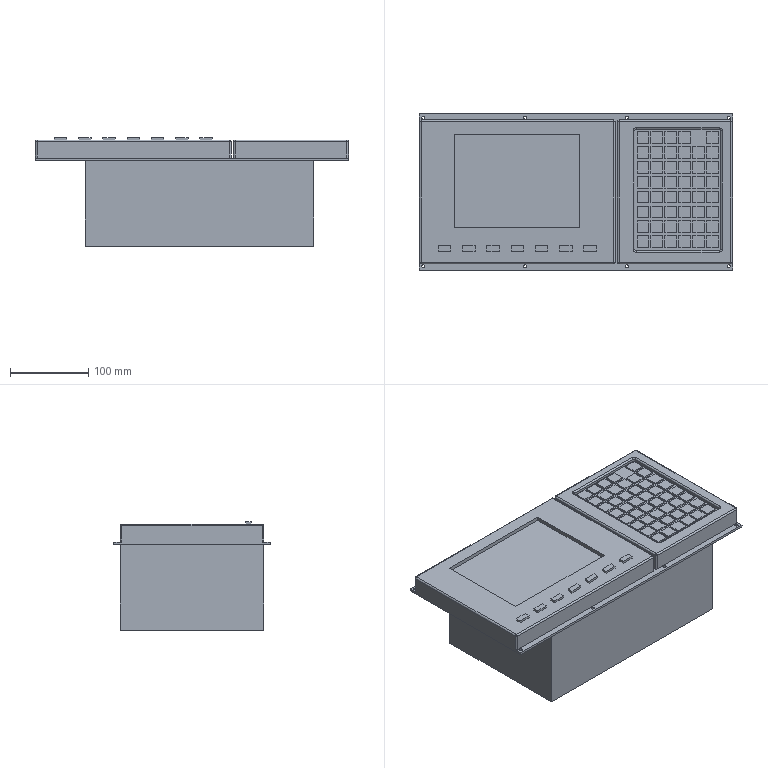Component | SolidWorks | ControlAssembly-1_System-2 | 1 solid | 351 faces | box 400 x 200 x 138.73 mm | volume 7643162 mm3 | plane 299 | cylinder 40 | sphere 8 | torus 4 | commonest cylinder face diameters 4 x40
build123d program:
from build123d import *

# Parameters (mm, degrees)
SKETCH1_W           = 400
SKETCH1_H           = 200
SKETCH1_R           = 2
BOSS_EXTRUDE1_DEPTH = 3
SKETCH2_W           = 400
SKETCH2_H           = 184
BOSS_EXTRUDE2_DEPTH = 23
SKETCH3_W           = 291.457
SKETCH3_H           = 184
BOSS_EXTRUDE3_DEPTH = 109.7
SKETCH4_W           = 160
SKETCH4_H           = 120
SKETCH4_W_2         = 110
SKETCH4_H_2         = 155
CUT_EXTRUDE1_DEPTH  = 5
SKETCH5_W           = 3
SKETCH5_H           = 184
CUT_EXTRUDE2_DEPTH  = 23
FILLET1_R           = 2
SKETCH6_W           = 16
SKETCH6_H           = 7
BOSS_EXTRUDE4_DEPTH = 3
SKETCH7_W           = 15
SKETCH7_H           = 15
BOSS_EXTRUDE5_DEPTH = 2


with BuildPart() as part:
    # Sketch1 → Boss-Extrude1 (new body)
    with BuildSketch(Plane.XY):
        with Locations((127.764, -62.597)):
            Rectangle(SKETCH1_W, SKETCH1_H)
        with Locations((-67.236, 32.403)):
            Circle(SKETCH1_R, mode=Mode.SUBTRACT)
        with Locations((62.764, 32.403)):
            Circle(SKETCH1_R, mode=Mode.SUBTRACT)
        with Locations((192.764, 32.403)):
            Circle(SKETCH1_R, mode=Mode.SUBTRACT)
        with Locations((322.764, 32.403)):
            Circle(SKETCH1_R, mode=Mode.SUBTRACT)
        with Locations((322.764, -157.597)):
            Circle(SKETCH1_R, mode=Mode.SUBTRACT)
        with Locations((192.764, -157.597)):
            Circle(SKETCH1_R, mode=Mode.SUBTRACT)
        with Locations((62.764, -157.597)):
            Circle(SKETCH1_R, mode=Mode.SUBTRACT)
        with Locations((-67.236, -157.597)):
            Circle(SKETCH1_R, mode=Mode.SUBTRACT)
    extrude(amount=BOSS_EXTRUDE1_DEPTH)

    # Sketch2 → Boss-Extrude2 (add)
    with BuildSketch(Plane.XY.offset(3)):
        with Locations((127.764, -62.597)):
            Rectangle(SKETCH2_W, SKETCH2_H)
    extrude(amount=BOSS_EXTRUDE2_DEPTH)

    # Sketch3 → Boss-Extrude3 (add)
    with BuildSketch(Plane(origin=(0, 0, 0), x_dir=(-1, 0, 0), z_dir=(0, 0, -1))):
        with Locations((-137.359, -62.597)):
            Rectangle(SKETCH3_W, SKETCH3_H)
    extrude(amount=BOSS_EXTRUDE3_DEPTH)

    # Sketch4 → Cut-Extrude1 (cut)
    with BuildSketch(Plane.XY.offset(26)):
        with Locations((52.764, -48.597)):
            Rectangle(SKETCH4_W, SKETCH4_H)
        with Locations((257.764, -60.097)):
            Rectangle(SKETCH4_W_2, SKETCH4_H_2)
    extrude(amount=-CUT_EXTRUDE1_DEPTH, mode=Mode.SUBTRACT)

    # Sketch5 → Cut-Extrude2 (cut)
    with BuildSketch(Plane.XY.offset(26)):
        with Locations((179.264, -62.597)):
            Rectangle(SKETCH5_W, SKETCH5_H)
    extrude(amount=-CUT_EXTRUDE2_DEPTH, mode=Mode.SUBTRACT)

    # Fillet1
    fillet1_edges = [part.edges().sort_by_distance(p)[0] for p in [
        (52.764, -154.597, 26),
        (-72.236, -62.597, 26),
        (52.764, 29.403, 26),
        (177.764, -62.597, 26),
        (312.764, -137.597, 23.5),
        (257.764, -137.597, 26),
        (202.764, -137.597, 23.5),
        (202.764, -60.097, 26),
        (202.764, 17.403, 23.5),
        (257.764, 17.403, 26),
        (312.764, 17.403, 23.5),
        (312.764, -60.097, 26),
        (177.764, 29.403, 14.5),
        (180.764, 29.403, 14.5),
        (254.264, 29.403, 26),
        (327.764, 29.403, 14.5),
        (327.764, -62.597, 26),
        (327.764, -154.597, 14.5),
        (254.264, -154.597, 26),
        (180.764, -62.597, 26),
        (180.764, -154.597, 14.5),
        (177.764, -154.597, 14.5),
        (-72.236, -154.597, 14.5),
        (-72.236, 29.403, 14.5),
    ]]
    fillet(fillet1_edges, radius=FILLET1_R)

    # Sketch6 → Boss-Extrude4 (add)
    with BuildSketch(Plane.XY.offset(26)):
        with Locations((-40.236, -134.676)):
            Rectangle(SKETCH6_W, SKETCH6_H)
        with Locations((-9.236, -134.676)):
            Rectangle(SKETCH6_W, SKETCH6_H)
        with Locations((21.764, -134.676)):
            Rectangle(SKETCH6_W, SKETCH6_H)
        with Locations((52.764, -134.676)):
            Rectangle(SKETCH6_W, SKETCH6_H)
        with Locations((83.764, -134.676)):
            Rectangle(SKETCH6_W, SKETCH6_H)
        with Locations((114.764, -134.676)):
            Rectangle(SKETCH6_W, SKETCH6_H)
        with Locations((145.764, -134.676)):
            Rectangle(SKETCH6_W, SKETCH6_H)
    extrude(amount=BOSS_EXTRUDE4_DEPTH)

    # Sketch7 → Boss-Extrude5 (add)
    with BuildSketch(Plane.XY.offset(21)):
        with Locations((213.264, 6.903)):
            Rectangle(SKETCH7_W, SKETCH7_H)
        with Locations((231.064, 6.903)):
            Rectangle(SKETCH7_W, SKETCH7_H)
        with Locations((248.864, 6.903)):
            Rectangle(SKETCH7_W, SKETCH7_H)
        with Locations((266.664, 6.903)):
            Rectangle(SKETCH7_W, SKETCH7_H)
        with Locations((302.264, 6.903)):
            Rectangle(SKETCH7_W, SKETCH7_H)
        with Locations((231.064, -12.097)):
            Rectangle(SKETCH7_W, SKETCH7_H)
        with Locations((248.864, -12.097)):
            Rectangle(SKETCH7_W, SKETCH7_H)
        with Locations((266.664, -12.097)):
            Rectangle(SKETCH7_W, SKETCH7_H)
        with Locations((284.464, -12.097)):
            Rectangle(SKETCH7_W, SKETCH7_H)
        with Locations((302.264, -12.097)):
            Rectangle(SKETCH7_W, SKETCH7_H)
        with Locations((231.064, -31.097)):
            Rectangle(SKETCH7_W, SKETCH7_H)
        with Locations((248.864, -31.097)):
            Rectangle(SKETCH7_W, SKETCH7_H)
        with Locations((266.664, -31.097)):
            Rectangle(SKETCH7_W, SKETCH7_H)
        with Locations((284.464, -31.097)):
            Rectangle(SKETCH7_W, SKETCH7_H)
        with Locations((302.264, -31.097)):
            Rectangle(SKETCH7_W, SKETCH7_H)
        with Locations((231.064, -50.097)):
            Rectangle(SKETCH7_W, SKETCH7_H)
        with Locations((248.864, -50.097)):
            Rectangle(SKETCH7_W, SKETCH7_H)
        with Locations((266.664, -50.097)):
            Rectangle(SKETCH7_W, SKETCH7_H)
        with Locations((284.464, -50.097)):
            Rectangle(SKETCH7_W, SKETCH7_H)
        with Locations((302.264, -50.097)):
            Rectangle(SKETCH7_W, SKETCH7_H)
        with Locations((231.064, -69.097)):
            Rectangle(SKETCH7_W, SKETCH7_H)
        with Locations((248.864, -69.097)):
            Rectangle(SKETCH7_W, SKETCH7_H)
        with Locations((266.664, -69.097)):
            Rectangle(SKETCH7_W, SKETCH7_H)
        with Locations((284.464, -69.097)):
            Rectangle(SKETCH7_W, SKETCH7_H)
        with Locations((302.264, -69.097)):
            Rectangle(SKETCH7_W, SKETCH7_H)
        with Locations((231.064, -88.097)):
            Rectangle(SKETCH7_W, SKETCH7_H)
        with Locations((248.864, -88.097)):
            Rectangle(SKETCH7_W, SKETCH7_H)
        with Locations((266.664, -88.097)):
            Rectangle(SKETCH7_W, SKETCH7_H)
        with Locations((284.464, -88.097)):
            Rectangle(SKETCH7_W, SKETCH7_H)
        with Locations((302.264, -88.097)):
            Rectangle(SKETCH7_W, SKETCH7_H)
        with Locations((231.064, -107.097)):
            Rectangle(SKETCH7_W, SKETCH7_H)
        with Locations((248.864, -107.097)):
            Rectangle(SKETCH7_W, SKETCH7_H)
        with Locations((266.664, -107.097)):
            Rectangle(SKETCH7_W, SKETCH7_H)
        with Locations((284.464, -107.097)):
            Rectangle(SKETCH7_W, SKETCH7_H)
        with Locations((302.264, -107.097)):
            Rectangle(SKETCH7_W, SKETCH7_H)
        with Locations((231.064, -126.097)):
            Rectangle(SKETCH7_W, SKETCH7_H)
        with Locations((248.864, -126.097)):
            Rectangle(SKETCH7_W, SKETCH7_H)
        with Locations((266.664, -126.097)):
            Rectangle(SKETCH7_W, SKETCH7_H)
        with Locations((284.464, -126.097)):
            Rectangle(SKETCH7_W, SKETCH7_H)
        with Locations((302.264, -126.097)):
            Rectangle(SKETCH7_W, SKETCH7_H)
        with Locations((213.264, -12.097)):
            Rectangle(SKETCH7_W, SKETCH7_H)
        with Locations((213.264, -31.097)):
            Rectangle(SKETCH7_W, SKETCH7_H)
        with Locations((213.264, -50.097)):
            Rectangle(SKETCH7_W, SKETCH7_H)
        with Locations((213.264, -69.097)):
            Rectangle(SKETCH7_W, SKETCH7_H)
        with Locations((213.264, -88.097)):
            Rectangle(SKETCH7_W, SKETCH7_H)
        with Locations((213.264, -107.097)):
            Rectangle(SKETCH7_W, SKETCH7_H)
        with Locations((213.264, -126.097)):
            Rectangle(SKETCH7_W, SKETCH7_H)
    extrude(amount=BOSS_EXTRUDE5_DEPTH)


solid = part.part

# Placed as in the assembly
solid = solid.moved(Location((437.691, 416.163, 511.468), (0, 0.005652, 0)))